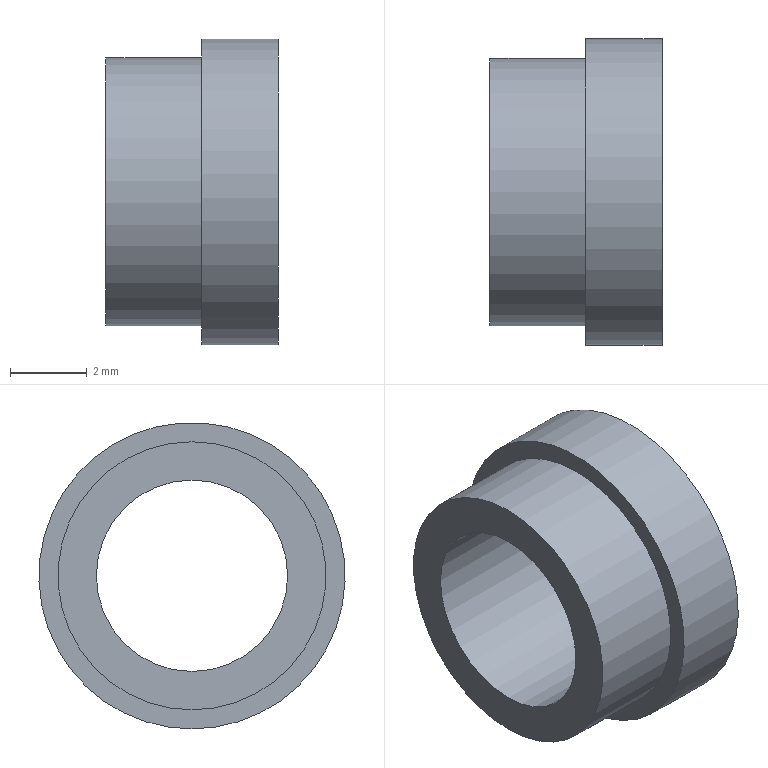Component | NX | END_CAP_3_BUSHING | 1 solid | 6 faces | volume 108 mm3 | plane 3 | cylinder 3 | commonest cylinder face diameters 7 x1 8 x1 5 x1